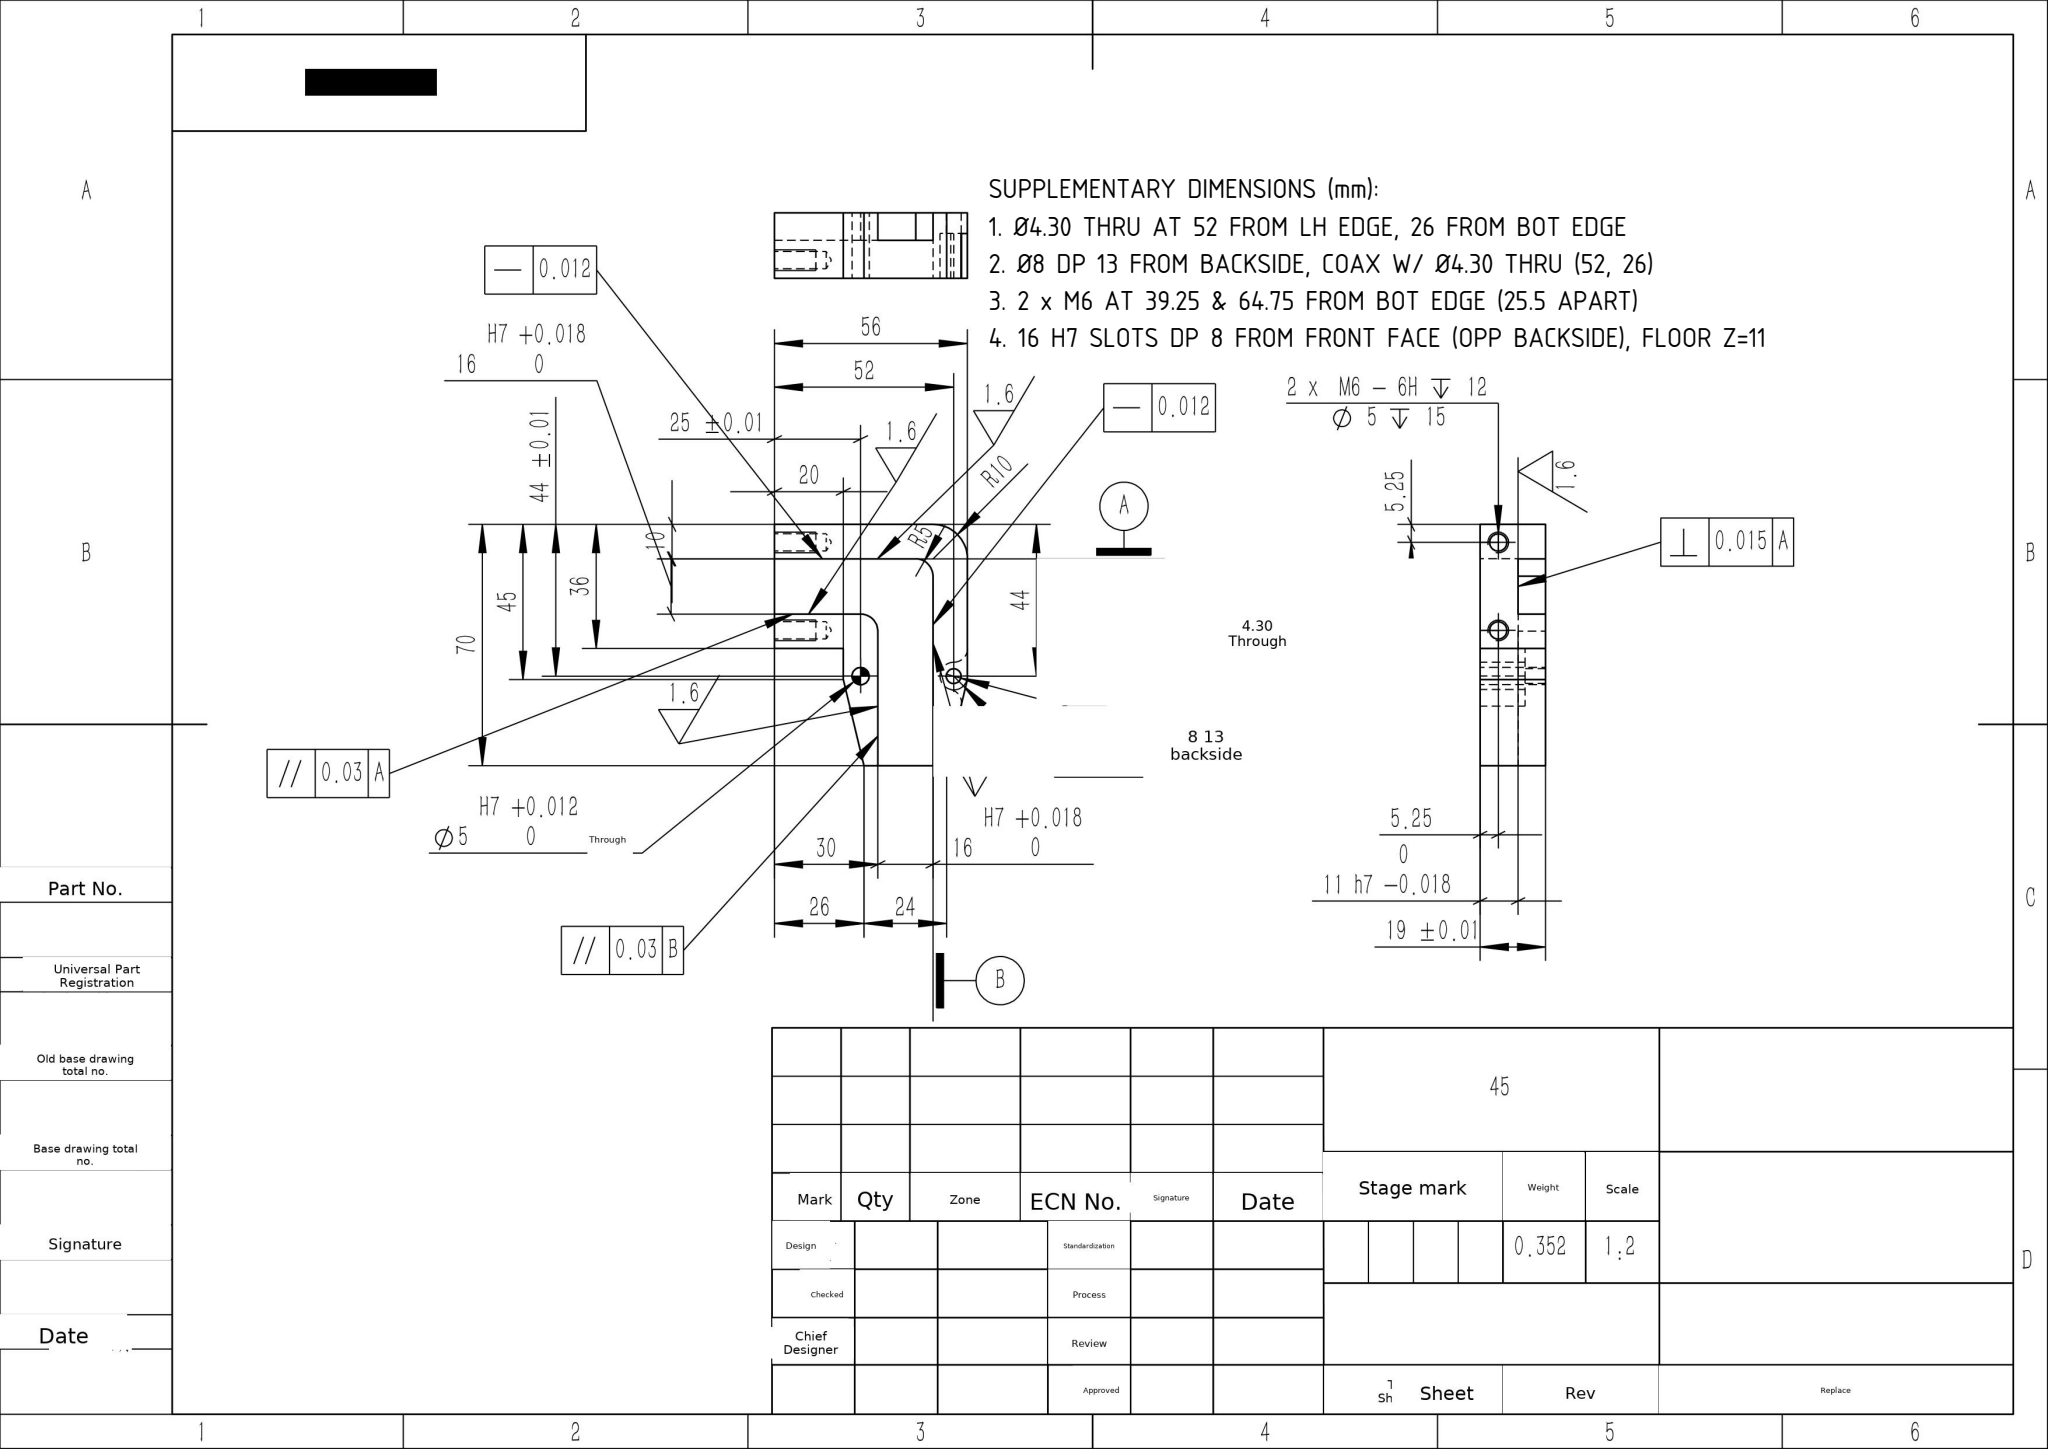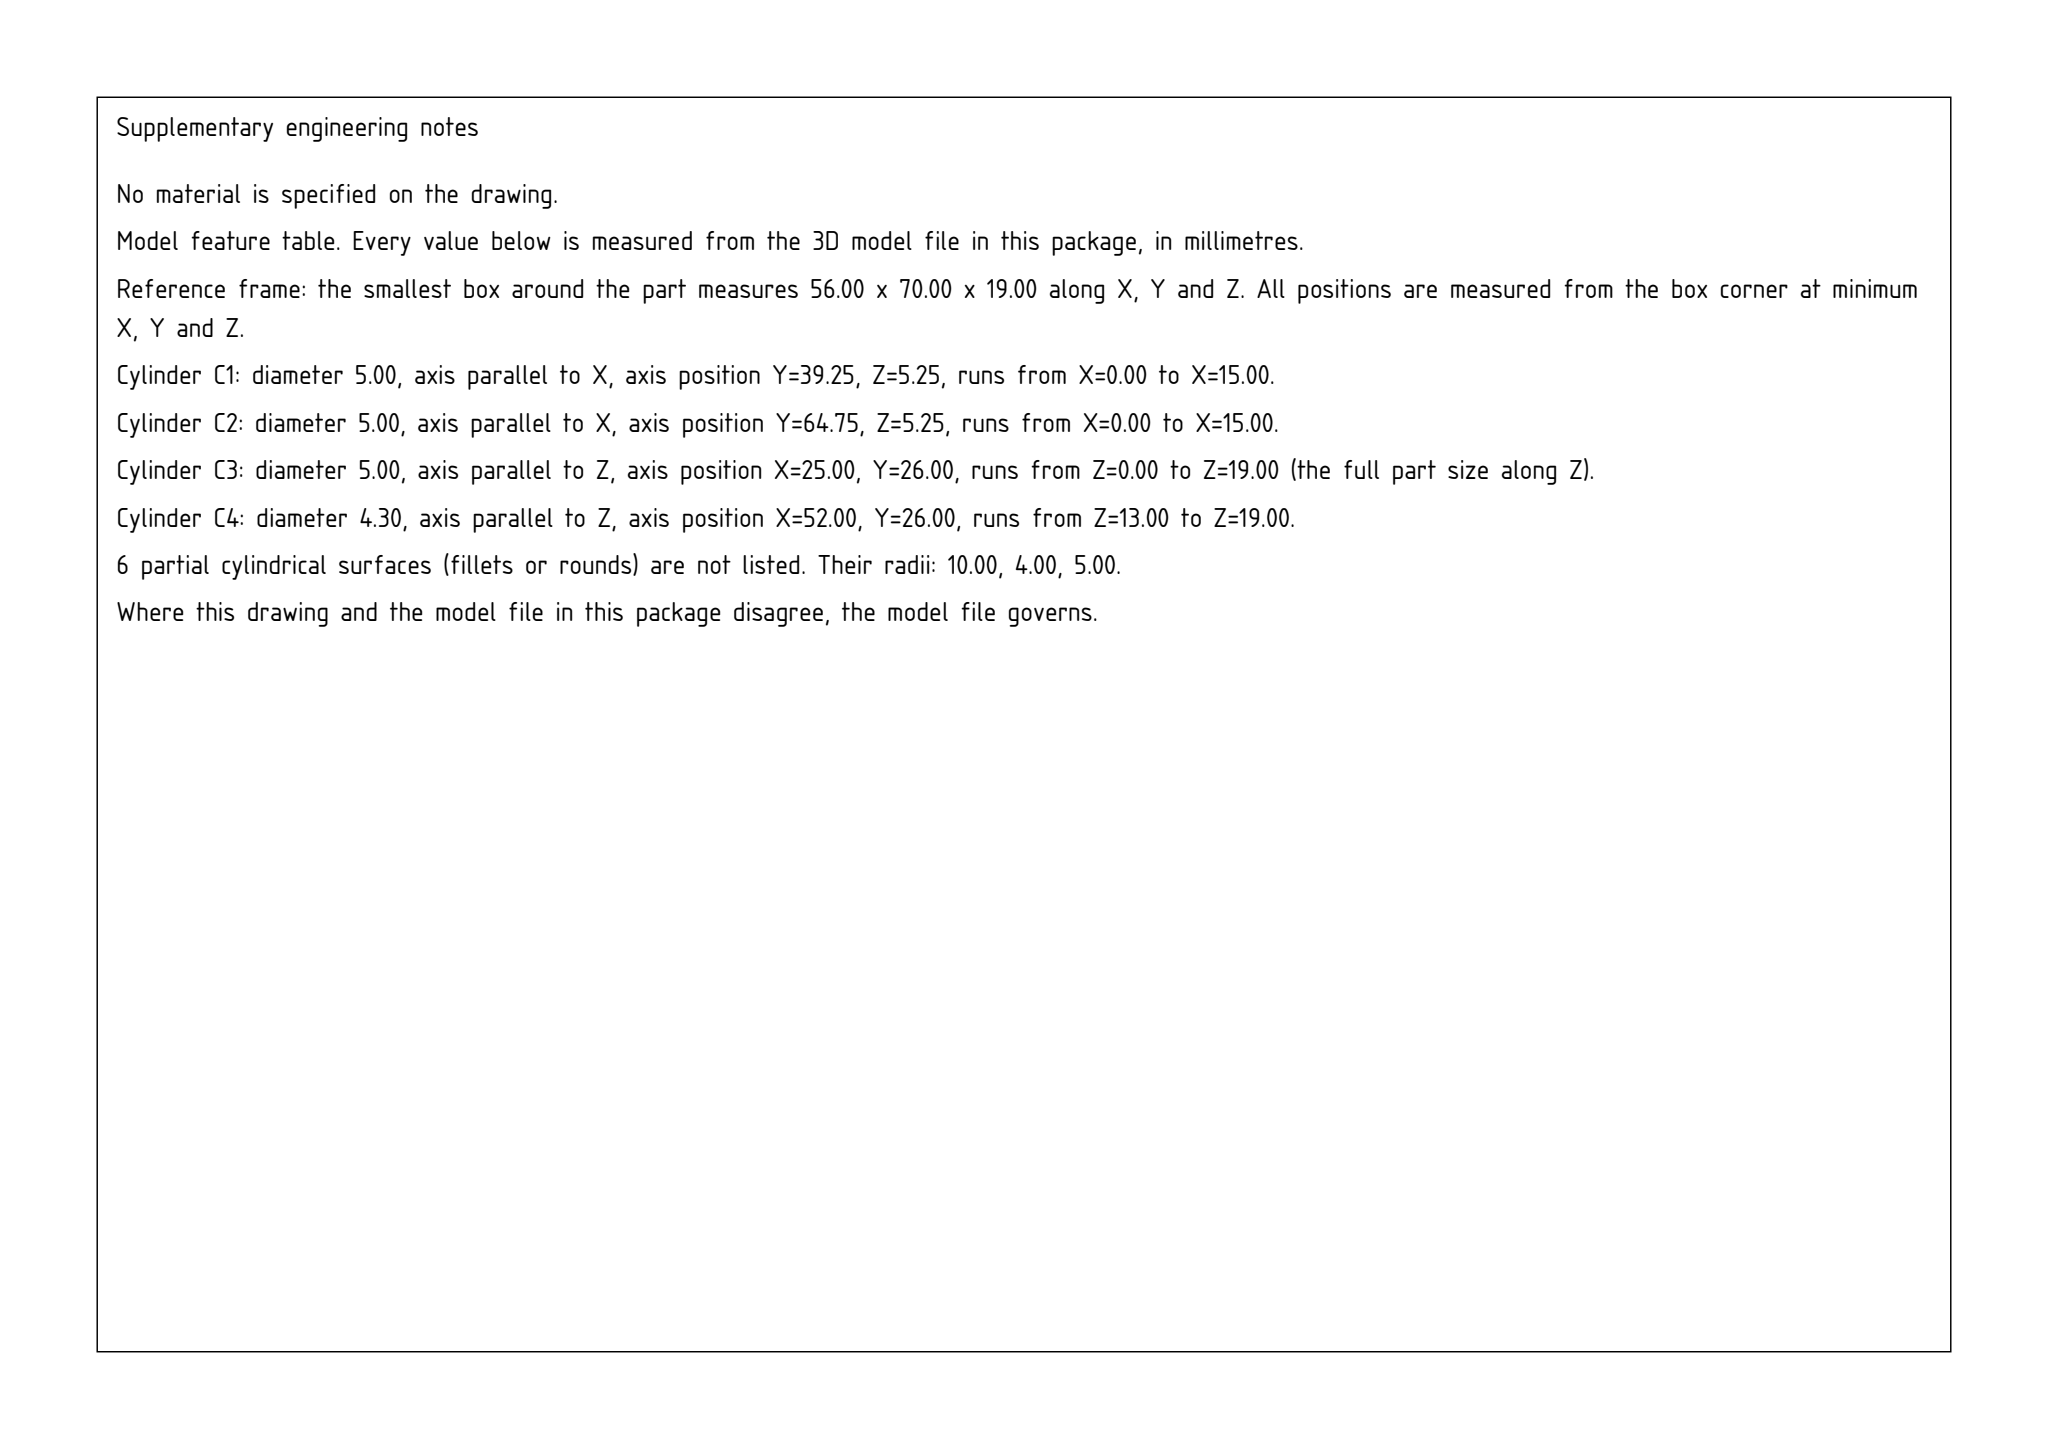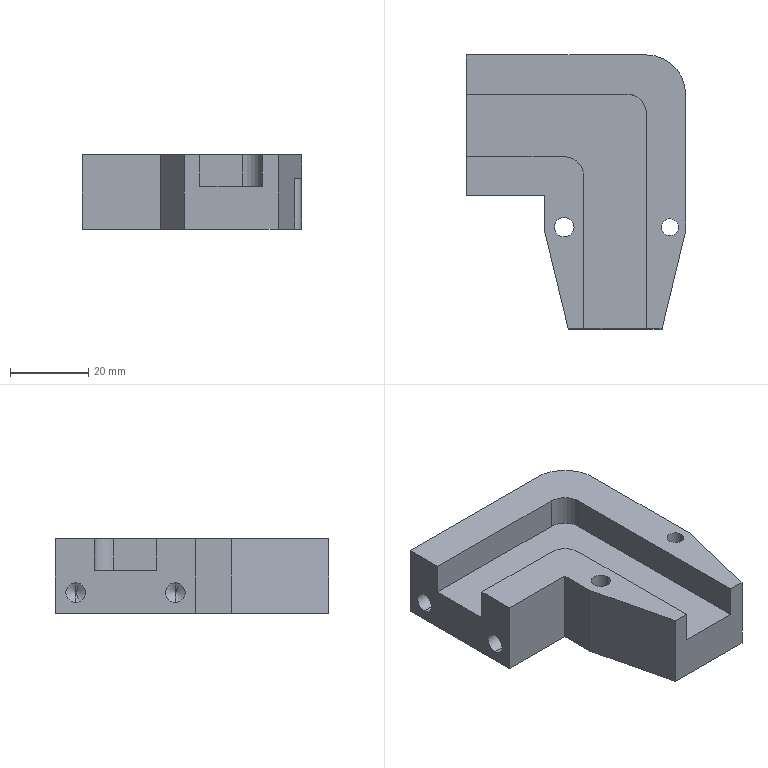Part | SolidWorks | mm | 1 solid | 37 faces | box 56 x 70 x 19 mm | volume 44875 mm3 | plane 17 | cylinder 16 | cone 4 | commonest cylinder face diameters 5 x6 8 x5 4.3 x2 10 x2 20 x1